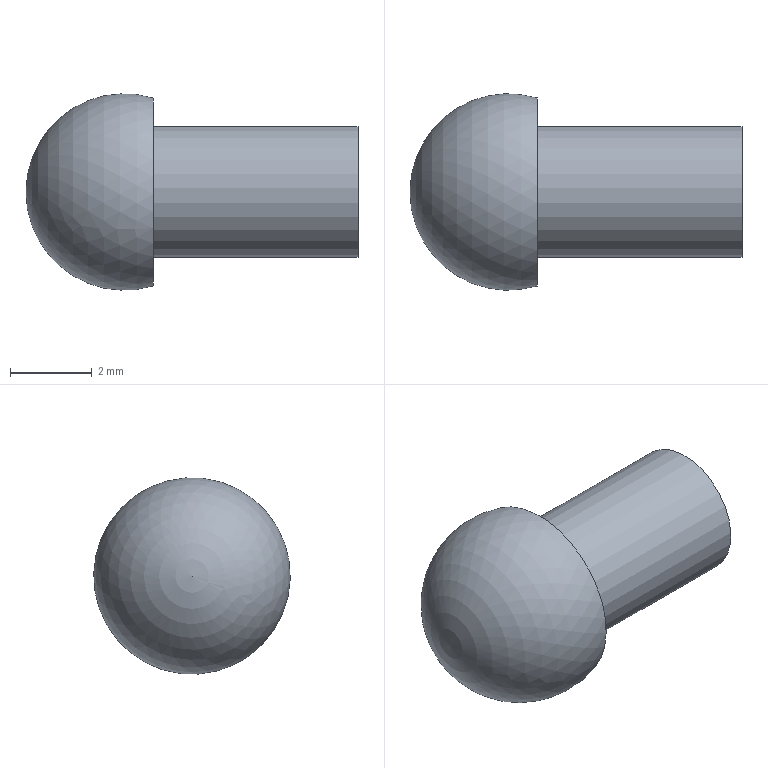Component | NX | VALVE_BALL | 1 solid | 4 faces | box 8.1 x 4.8 x 4.8 mm | volume 81 mm3 | plane 2 | cylinder 1 | sphere 1 | commonest cylinder face diameters 3.2 x1
STEP:
#1=CARTESIAN_POINT('',(0.,0.,0.));
#2=DIRECTION('',(0.,0.,1.));
#3=DIRECTION('',(1.,0.,0.));
#4=AXIS2_PLACEMENT_3D('',#1,#2,#3);
#5=CARTESIAN_POINT('',(33.094,50.479,-0.389));
#6=VERTEX_POINT('',#5);
#7=CARTESIAN_POINT('',(33.094,49.,-1.));
#8=DIRECTION('',(-1.,0.,0.));
#9=DIRECTION('',(0.,0.9242,0.3818));
#10=AXIS2_PLACEMENT_3D('',#7,#8,#9);
#11=CIRCLE('',#10,1.6);
#12=CARTESIAN_POINT('',(38.094,49.,-1.));
#13=DIRECTION('',(-1.,0.,0.));
#14=DIRECTION('',(0.,0.9242,0.3818));
#15=AXIS2_PLACEMENT_3D('',#12,#13,#14);
#16=CYLINDRICAL_SURFACE('',#15,1.6);
#17=CARTESIAN_POINT('',(0.,5.));
#18=DIRECTION('',(1.,0.));
#19=VECTOR('',#18,1.);
#20=LINE('',#17,#19);
#21=(GEOMETRIC_REPRESENTATION_CONTEXT(2)PARAMETRIC_REPRESENTATION_CONTEXT()REPRESENTATION_CONTEXT('',''));
#22=DEFINITIONAL_REPRESENTATION('',(#20),#21);
#23=PCURVE('',#16,#22);
#24=CARTESIAN_POINT('',(33.094,47.521,-1.611));
#25=DIRECTION('',(-1.,0.,0.));
#26=DIRECTION('',(0.,0.9242,0.3818));
#27=AXIS2_PLACEMENT_3D('',#24,#25,#26);
#28=PLANE('',#27);
#29=CARTESIAN_POINT('',(1.6,0.));
#30=DIRECTION('',(1.,0.));
#31=AXIS2_PLACEMENT_2D('',#29,#30);
#32=CIRCLE('',#31,1.6);
#33=(GEOMETRIC_REPRESENTATION_CONTEXT(2)PARAMETRIC_REPRESENTATION_CONTEXT()REPRESENTATION_CONTEXT('',''));
#34=DEFINITIONAL_REPRESENTATION('',(#32),#33);
#35=PCURVE('',#28,#34);
#36=SURFACE_CURVE('',#11,(#23,#35),.PCURVE_S1.);
#37=EDGE_CURVE('',#6,#6,#36,.T.);
#38=ORIENTED_EDGE('',*,*,#37,.F.);
#39=CARTESIAN_POINT('',(38.094,50.479,-0.389));
#40=VERTEX_POINT('',#39);
#41=CARTESIAN_POINT('',(38.094,50.479,-0.389));
#42=CARTESIAN_POINT('',(33.094,50.479,-0.389));
#43=B_SPLINE_CURVE_WITH_KNOTS('',1,(#41,#42),.UNSPECIFIED.,.F.,.F.,(2,2),(0.,5.),.PIECEWISE_BEZIER_KNOTS.);
#44=CARTESIAN_POINT('',(0.,0.));
#45=DIRECTION('',(0.,1.));
#46=VECTOR('',#45,1.);
#47=LINE('',#44,#46);
#48=(GEOMETRIC_REPRESENTATION_CONTEXT(2)PARAMETRIC_REPRESENTATION_CONTEXT()REPRESENTATION_CONTEXT('',''));
#49=DEFINITIONAL_REPRESENTATION('',(#47),#48);
#50=PCURVE('',#16,#49);
#51=CARTESIAN_POINT('',(6.283,0.));
#52=DIRECTION('',(0.,1.));
#53=VECTOR('',#52,1.);
#54=LINE('',#51,#53);
#55=(GEOMETRIC_REPRESENTATION_CONTEXT(2)PARAMETRIC_REPRESENTATION_CONTEXT()REPRESENTATION_CONTEXT('',''));
#56=DEFINITIONAL_REPRESENTATION('',(#54),#55);
#57=PCURVE('',#16,#56);
#58=SEAM_CURVE('',#43,(#50,#57),.PCURVE_S1.);
#59=EDGE_CURVE('',#40,#6,#58,.T.);
#60=ORIENTED_EDGE('',*,*,#59,.F.);
#61=CARTESIAN_POINT('',(38.094,49.,-1.));
#62=DIRECTION('',(-1.,0.,0.));
#63=DIRECTION('',(0.,0.9242,0.3818));
#64=AXIS2_PLACEMENT_3D('',#61,#62,#63);
#65=CIRCLE('',#64,1.6);
#66=CARTESIAN_POINT('',(0.,0.));
#67=DIRECTION('',(1.,0.));
#68=VECTOR('',#67,1.);
#69=LINE('',#66,#68);
#70=(GEOMETRIC_REPRESENTATION_CONTEXT(2)PARAMETRIC_REPRESENTATION_CONTEXT()REPRESENTATION_CONTEXT('',''));
#71=DEFINITIONAL_REPRESENTATION('',(#69),#70);
#72=PCURVE('',#16,#71);
#73=CARTESIAN_POINT('',(38.094,49.,-1.));
#74=DIRECTION('',(-1.,0.,0.));
#75=DIRECTION('',(0.,0.9242,0.3818));
#76=AXIS2_PLACEMENT_3D('',#73,#74,#75);
#77=PLANE('',#76);
#78=CARTESIAN_POINT('',(0.,0.));
#79=DIRECTION('',(1.,0.));
#80=AXIS2_PLACEMENT_2D('',#78,#79);
#81=CIRCLE('',#80,1.6);
#82=(GEOMETRIC_REPRESENTATION_CONTEXT(2)PARAMETRIC_REPRESENTATION_CONTEXT()REPRESENTATION_CONTEXT('',''));
#83=DEFINITIONAL_REPRESENTATION('',(#81),#82);
#84=PCURVE('',#77,#83);
#85=SURFACE_CURVE('',#65,(#72,#84),.PCURVE_S1.);
#86=EDGE_CURVE('',#40,#40,#85,.T.);
#87=ORIENTED_EDGE('',*,*,#86,.T.);
#88=ORIENTED_EDGE('',*,*,#59,.T.);
#89=EDGE_LOOP('',(#38,#60,#87,#88));
#90=FACE_BOUND('',#89,.T.);
#91=ADVANCED_FACE('',(#90),#16,.T.);
#92=CARTESIAN_POINT('',(33.094,51.122,-0.1234));
#93=VERTEX_POINT('',#92);
#94=CARTESIAN_POINT('',(33.094,46.878,-1.877));
#95=VERTEX_POINT('',#94);
#96=CARTESIAN_POINT('',(33.094,49.,-1.));
#97=DIRECTION('',(-1.,0.,0.));
#98=DIRECTION('',(0.,0.9242,0.3818));
#99=AXIS2_PLACEMENT_3D('',#96,#97,#98);
#100=CIRCLE('',#99,2.296);
#101=CARTESIAN_POINT('',(1.6,0.));
#102=DIRECTION('',(1.,-0.));
#103=AXIS2_PLACEMENT_2D('',#101,#102);
#104=CIRCLE('',#103,2.296);
#105=(GEOMETRIC_REPRESENTATION_CONTEXT(2)PARAMETRIC_REPRESENTATION_CONTEXT()REPRESENTATION_CONTEXT('',''));
#106=DEFINITIONAL_REPRESENTATION('',(#104),#105);
#107=PCURVE('',#28,#106);
#108=CARTESIAN_POINT('',(32.394,49.,-1.));
#109=DIRECTION('',(-1.,0.,0.));
#110=DIRECTION('',(0.,-0.9242,-0.3818));
#111=AXIS2_PLACEMENT_3D('',#108,#109,#110);
#112=SPHERICAL_SURFACE('',#111,2.4);
#113=CARTESIAN_POINT('',(3.142,-0.296));
#114=CARTESIAN_POINT('',(3.237,-0.296));
#115=CARTESIAN_POINT('',(3.427,-0.296));
#116=CARTESIAN_POINT('',(3.713,-0.296));
#117=CARTESIAN_POINT('',(3.998,-0.296));
#118=CARTESIAN_POINT('',(4.284,-0.296));
#119=CARTESIAN_POINT('',(4.57,-0.296));
#120=CARTESIAN_POINT('',(4.855,-0.296));
#121=CARTESIAN_POINT('',(5.141,-0.296));
#122=CARTESIAN_POINT('',(5.426,-0.296));
#123=CARTESIAN_POINT('',(5.712,-0.296));
#124=CARTESIAN_POINT('',(5.998,-0.296));
#125=CARTESIAN_POINT('',(6.283,-0.296));
#126=CARTESIAN_POINT('',(6.569,-0.296));
#127=CARTESIAN_POINT('',(6.854,-0.296));
#128=CARTESIAN_POINT('',(7.14,-0.296));
#129=CARTESIAN_POINT('',(7.426,-0.296));
#130=CARTESIAN_POINT('',(7.711,-0.296));
#131=CARTESIAN_POINT('',(7.997,-0.296));
#132=CARTESIAN_POINT('',(8.282,-0.296));
#133=CARTESIAN_POINT('',(8.568,-0.296));
#134=CARTESIAN_POINT('',(8.854,-0.296));
#135=CARTESIAN_POINT('',(9.139,-0.296));
#136=CARTESIAN_POINT('',(9.33,-0.296));
#137=CARTESIAN_POINT('',(9.425,-0.296));
#138=B_SPLINE_CURVE_WITH_KNOTS('',3,(#113,#114,#115,#116,#117,#118,#119,#120,#121,#122,#123,#124,#125,#126,#127,#128,#129,#130,#131,#132,#133,#134,#135,#136,#137),.UNSPECIFIED.,.F.,.F.,(4,1,1,1,1,1,1,1,1,1,1,1,1,1,1,1,1,1,1,1,1,1,4),(0.,0.2856,0.5712,0.8568,1.142,1.428,1.714,1.999,2.285,2.57,2.856,3.142,3.427,3.713,3.998,4.284,4.57,4.855,5.141,5.426,5.712,5.998,6.283),.QUASI_UNIFORM_KNOTS.);
#139=(GEOMETRIC_REPRESENTATION_CONTEXT(2)PARAMETRIC_REPRESENTATION_CONTEXT()REPRESENTATION_CONTEXT('',''));
#140=DEFINITIONAL_REPRESENTATION('',(#138),#139);
#141=PCURVE('',#112,#140);
#142=SURFACE_CURVE('',#100,(#107,#141),.PCURVE_S1.);
#143=EDGE_CURVE('',#93,#95,#142,.T.);
#144=ORIENTED_EDGE('',*,*,#143,.F.);
#145=CARTESIAN_POINT('',(33.094,49.,-1.));
#146=DIRECTION('',(-1.,0.,0.));
#147=DIRECTION('',(0.,0.9242,0.3818));
#148=AXIS2_PLACEMENT_3D('',#145,#146,#147);
#149=CIRCLE('',#148,2.296);
#150=CARTESIAN_POINT('',(1.6,0.));
#151=DIRECTION('',(1.,-0.));
#152=AXIS2_PLACEMENT_2D('',#150,#151);
#153=CIRCLE('',#152,2.296);
#154=(GEOMETRIC_REPRESENTATION_CONTEXT(2)PARAMETRIC_REPRESENTATION_CONTEXT()REPRESENTATION_CONTEXT('',''));
#155=DEFINITIONAL_REPRESENTATION('',(#153),#154);
#156=PCURVE('',#28,#155);
#157=CARTESIAN_POINT('',(-3.142,-0.296));
#158=CARTESIAN_POINT('',(-3.046,-0.296));
#159=CARTESIAN_POINT('',(-2.856,-0.296));
#160=CARTESIAN_POINT('',(-2.57,-0.296));
#161=CARTESIAN_POINT('',(-2.285,-0.296));
#162=CARTESIAN_POINT('',(-1.999,-0.296));
#163=CARTESIAN_POINT('',(-1.714,-0.296));
#164=CARTESIAN_POINT('',(-1.428,-0.296));
#165=CARTESIAN_POINT('',(-1.142,-0.296));
#166=CARTESIAN_POINT('',(-0.8568,-0.296));
#167=CARTESIAN_POINT('',(-0.5712,-0.296));
#168=CARTESIAN_POINT('',(-0.2856,-0.296));
#169=CARTESIAN_POINT('',(-0.,-0.296));
#170=CARTESIAN_POINT('',(0.2856,-0.296));
#171=CARTESIAN_POINT('',(0.5712,-0.296));
#172=CARTESIAN_POINT('',(0.8568,-0.296));
#173=CARTESIAN_POINT('',(1.142,-0.296));
#174=CARTESIAN_POINT('',(1.428,-0.296));
#175=CARTESIAN_POINT('',(1.714,-0.296));
#176=CARTESIAN_POINT('',(1.999,-0.296));
#177=CARTESIAN_POINT('',(2.285,-0.296));
#178=CARTESIAN_POINT('',(2.57,-0.296));
#179=CARTESIAN_POINT('',(2.856,-0.296));
#180=CARTESIAN_POINT('',(3.046,-0.296));
#181=CARTESIAN_POINT('',(3.142,-0.296));
#182=B_SPLINE_CURVE_WITH_KNOTS('',3,(#157,#158,#159,#160,#161,#162,#163,#164,#165,#166,#167,#168,#169,#170,#171,#172,#173,#174,#175,#176,#177,#178,#179,#180,#181),.UNSPECIFIED.,.F.,.F.,(4,1,1,1,1,1,1,1,1,1,1,1,1,1,1,1,1,1,1,1,1,1,4),(0.,0.2856,0.5712,0.8568,1.142,1.428,1.714,1.999,2.285,2.57,2.856,3.142,3.427,3.713,3.998,4.284,4.57,4.855,5.141,5.426,5.712,5.998,6.283),.QUASI_UNIFORM_KNOTS.);
#183=(GEOMETRIC_REPRESENTATION_CONTEXT(2)PARAMETRIC_REPRESENTATION_CONTEXT()REPRESENTATION_CONTEXT('',''));
#184=DEFINITIONAL_REPRESENTATION('',(#182),#183);
#185=PCURVE('',#112,#184);
#186=SURFACE_CURVE('',#149,(#156,#185),.PCURVE_S1.);
#187=EDGE_CURVE('',#95,#93,#186,.T.);
#188=ORIENTED_EDGE('',*,*,#187,.F.);
#189=EDGE_LOOP('',(#144,#188));
#190=FACE_BOUND('',#189,.T.);
#191=ORIENTED_EDGE('',*,*,#37,.T.);
#192=EDGE_LOOP('',(#191));
#193=FACE_BOUND('',#192,.T.);
#194=ADVANCED_FACE('',(#190,#193),#28,.F.);
#195=ORIENTED_EDGE('',*,*,#143,.T.);
#196=CARTESIAN_POINT('',(29.994,49.,-1.));
#197=VERTEX_POINT('',#196);
#198=CARTESIAN_POINT('',(33.094,46.878,-1.877));
#199=CARTESIAN_POINT('',(32.482,46.706,-1.948));
#200=CARTESIAN_POINT('',(31.812,46.709,-1.946));
#201=CARTESIAN_POINT('',(31.154,46.909,-1.864));
#202=CARTESIAN_POINT('',(30.591,47.294,-1.705));
#203=CARTESIAN_POINT('',(30.193,47.817,-1.489));
#204=CARTESIAN_POINT('',(29.994,48.408,-1.244));
#205=CARTESIAN_POINT('',(29.994,49.,-1.));
#206=B_SPLINE_CURVE_WITH_KNOTS('',7,(#198,#199,#200,#201,#202,#203,#204,#205),.UNSPECIFIED.,.F.,.F.,(8,8),(-0.296,1.571),.PIECEWISE_BEZIER_KNOTS.);
#207=CARTESIAN_POINT('',(6.283,0.));
#208=DIRECTION('',(0.,1.));
#209=VECTOR('',#208,1.);
#210=LINE('',#207,#209);
#211=(GEOMETRIC_REPRESENTATION_CONTEXT(2)PARAMETRIC_REPRESENTATION_CONTEXT()REPRESENTATION_CONTEXT('',''));
#212=DEFINITIONAL_REPRESENTATION('',(#210),#211);
#213=PCURVE('',#112,#212);
#214=CARTESIAN_POINT('',(0.,0.));
#215=DIRECTION('',(0.,1.));
#216=VECTOR('',#215,1.);
#217=LINE('',#214,#216);
#218=(GEOMETRIC_REPRESENTATION_CONTEXT(2)PARAMETRIC_REPRESENTATION_CONTEXT()REPRESENTATION_CONTEXT('',''));
#219=DEFINITIONAL_REPRESENTATION('',(#217),#218);
#220=PCURVE('',#112,#219);
#221=SEAM_CURVE('',#206,(#213,#220),.PCURVE_S1.);
#222=EDGE_CURVE('',#95,#197,#221,.T.);
#223=ORIENTED_EDGE('',*,*,#222,.T.);
#224=ORIENTED_EDGE('',*,*,#222,.F.);
#225=ORIENTED_EDGE('',*,*,#187,.T.);
#226=EDGE_LOOP('',(#195,#223,#224,#225));
#227=FACE_BOUND('',#226,.T.);
#228=ADVANCED_FACE('',(#227),#112,.T.);
#229=ORIENTED_EDGE('',*,*,#86,.F.);
#230=EDGE_LOOP('',(#229));
#231=FACE_BOUND('',#230,.T.);
#232=ADVANCED_FACE('',(#231),#77,.F.);
#233=CLOSED_SHELL('',(#91,#194,#228,#232));
#234=MANIFOLD_SOLID_BREP('',#233);
#235=(LENGTH_UNIT()NAMED_UNIT(*)SI_UNIT(.MILLI.,.METRE.));
#236=UNCERTAINTY_MEASURE_WITH_UNIT(LENGTH_MEASURE(0.000005),#235,'','');
#237=(NAMED_UNIT(*)PLANE_ANGLE_UNIT()SI_UNIT($,.RADIAN.));
#238=(NAMED_UNIT(*)SI_UNIT($,.STERADIAN.)SOLID_ANGLE_UNIT());
#239=(GEOMETRIC_REPRESENTATION_CONTEXT(3)GLOBAL_UNCERTAINTY_ASSIGNED_CONTEXT((#236))GLOBAL_UNIT_ASSIGNED_CONTEXT((#235,#237,#238))REPRESENTATION_CONTEXT('',''));
#240=ADVANCED_BREP_SHAPE_REPRESENTATION('',(#4,#234),#239);